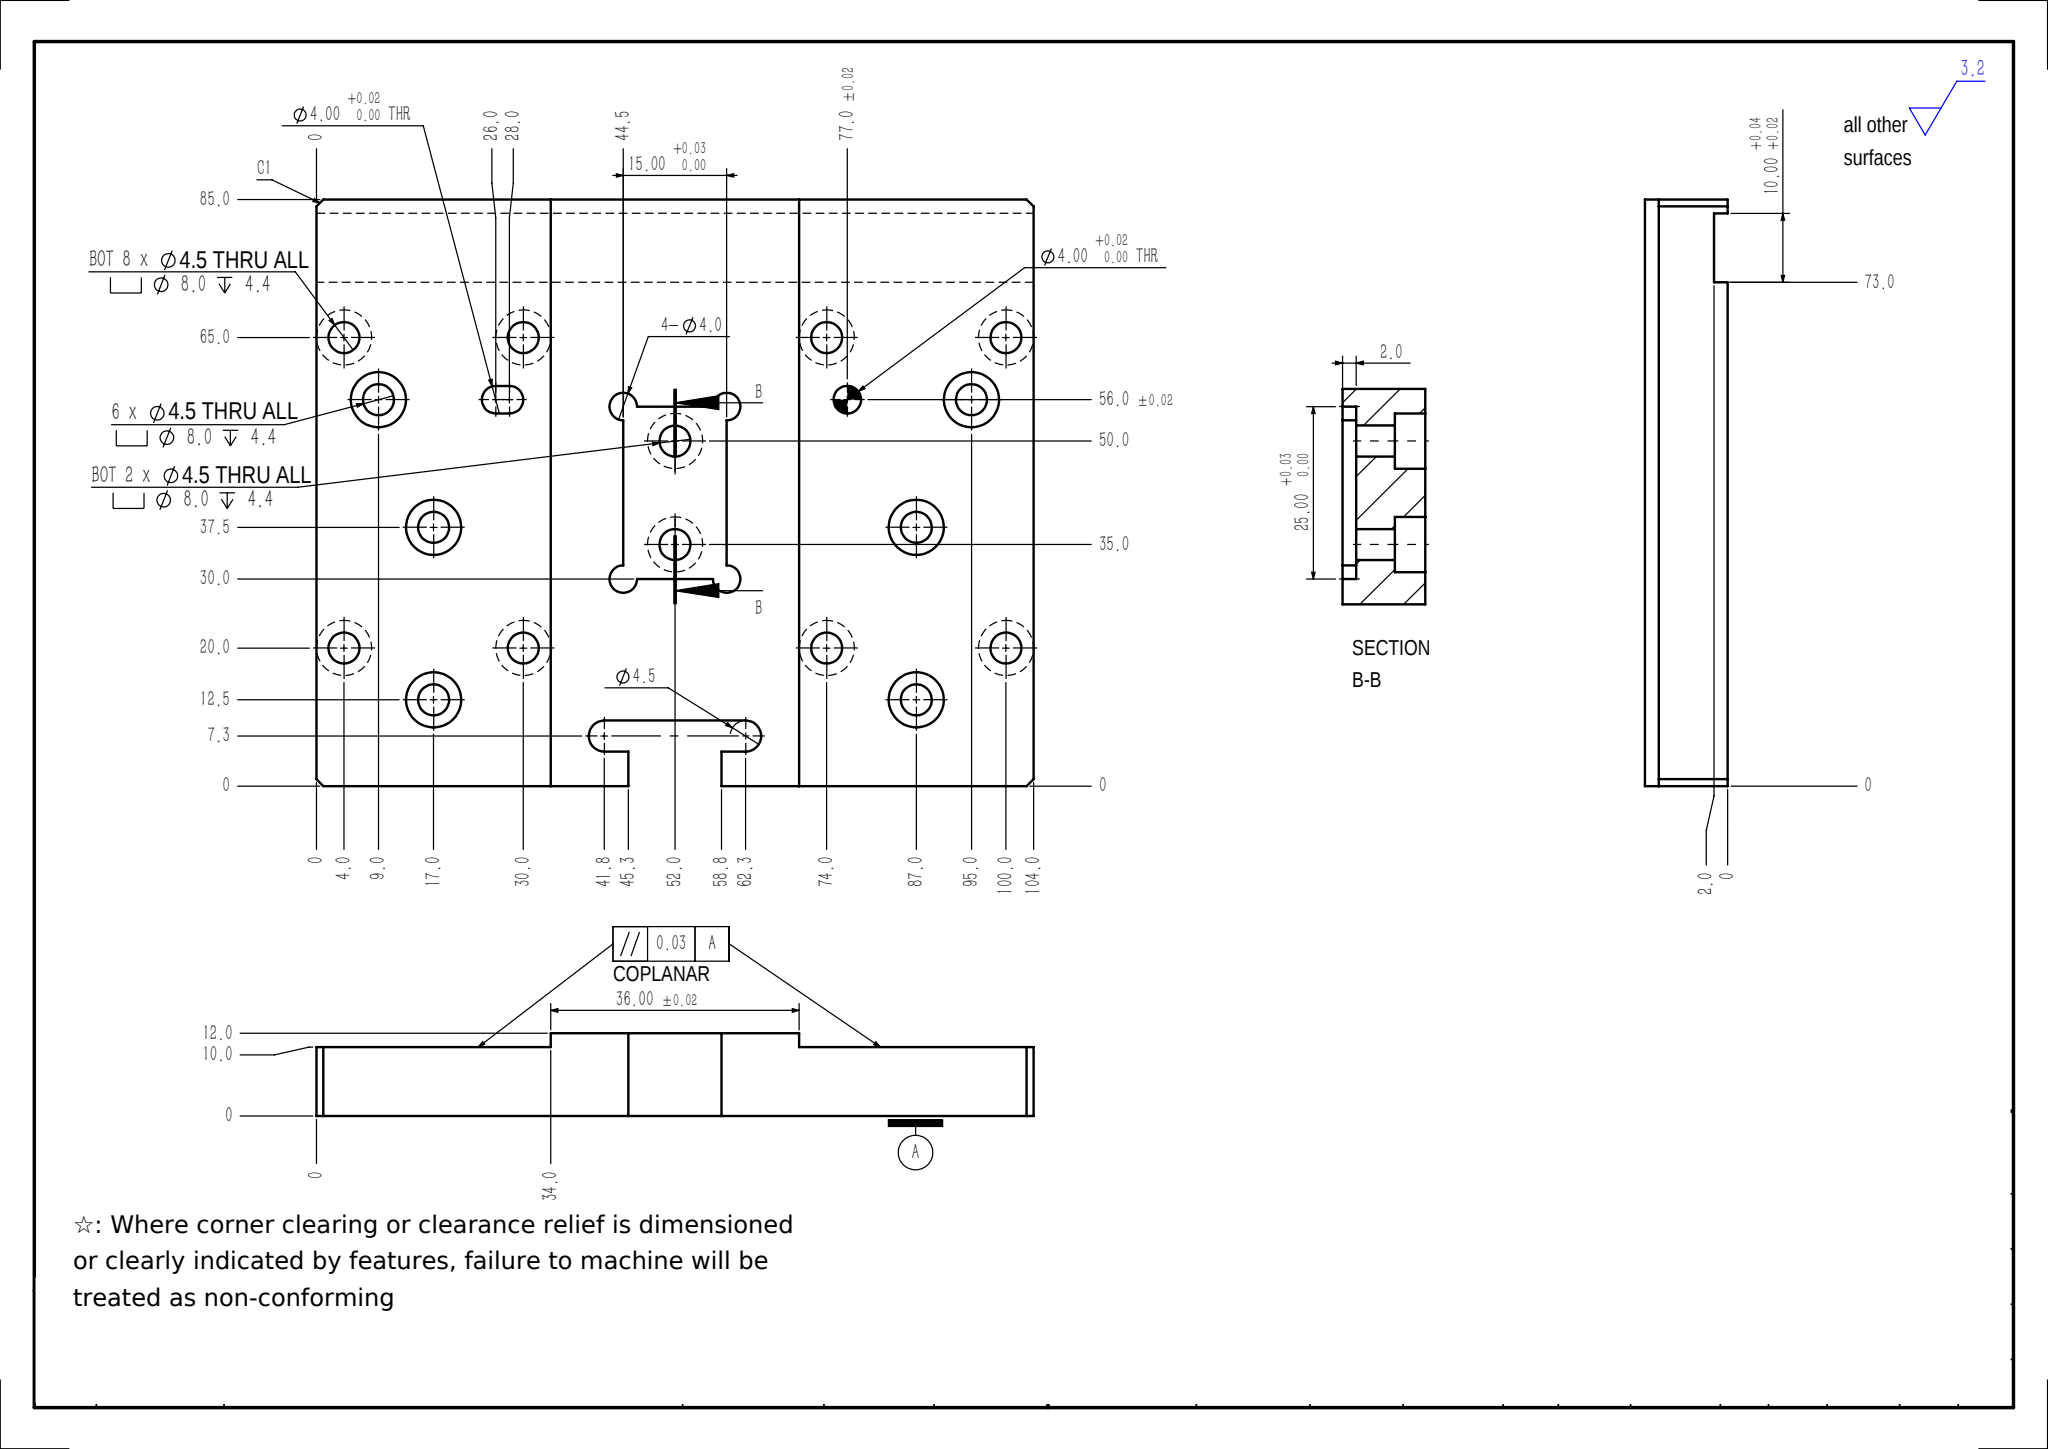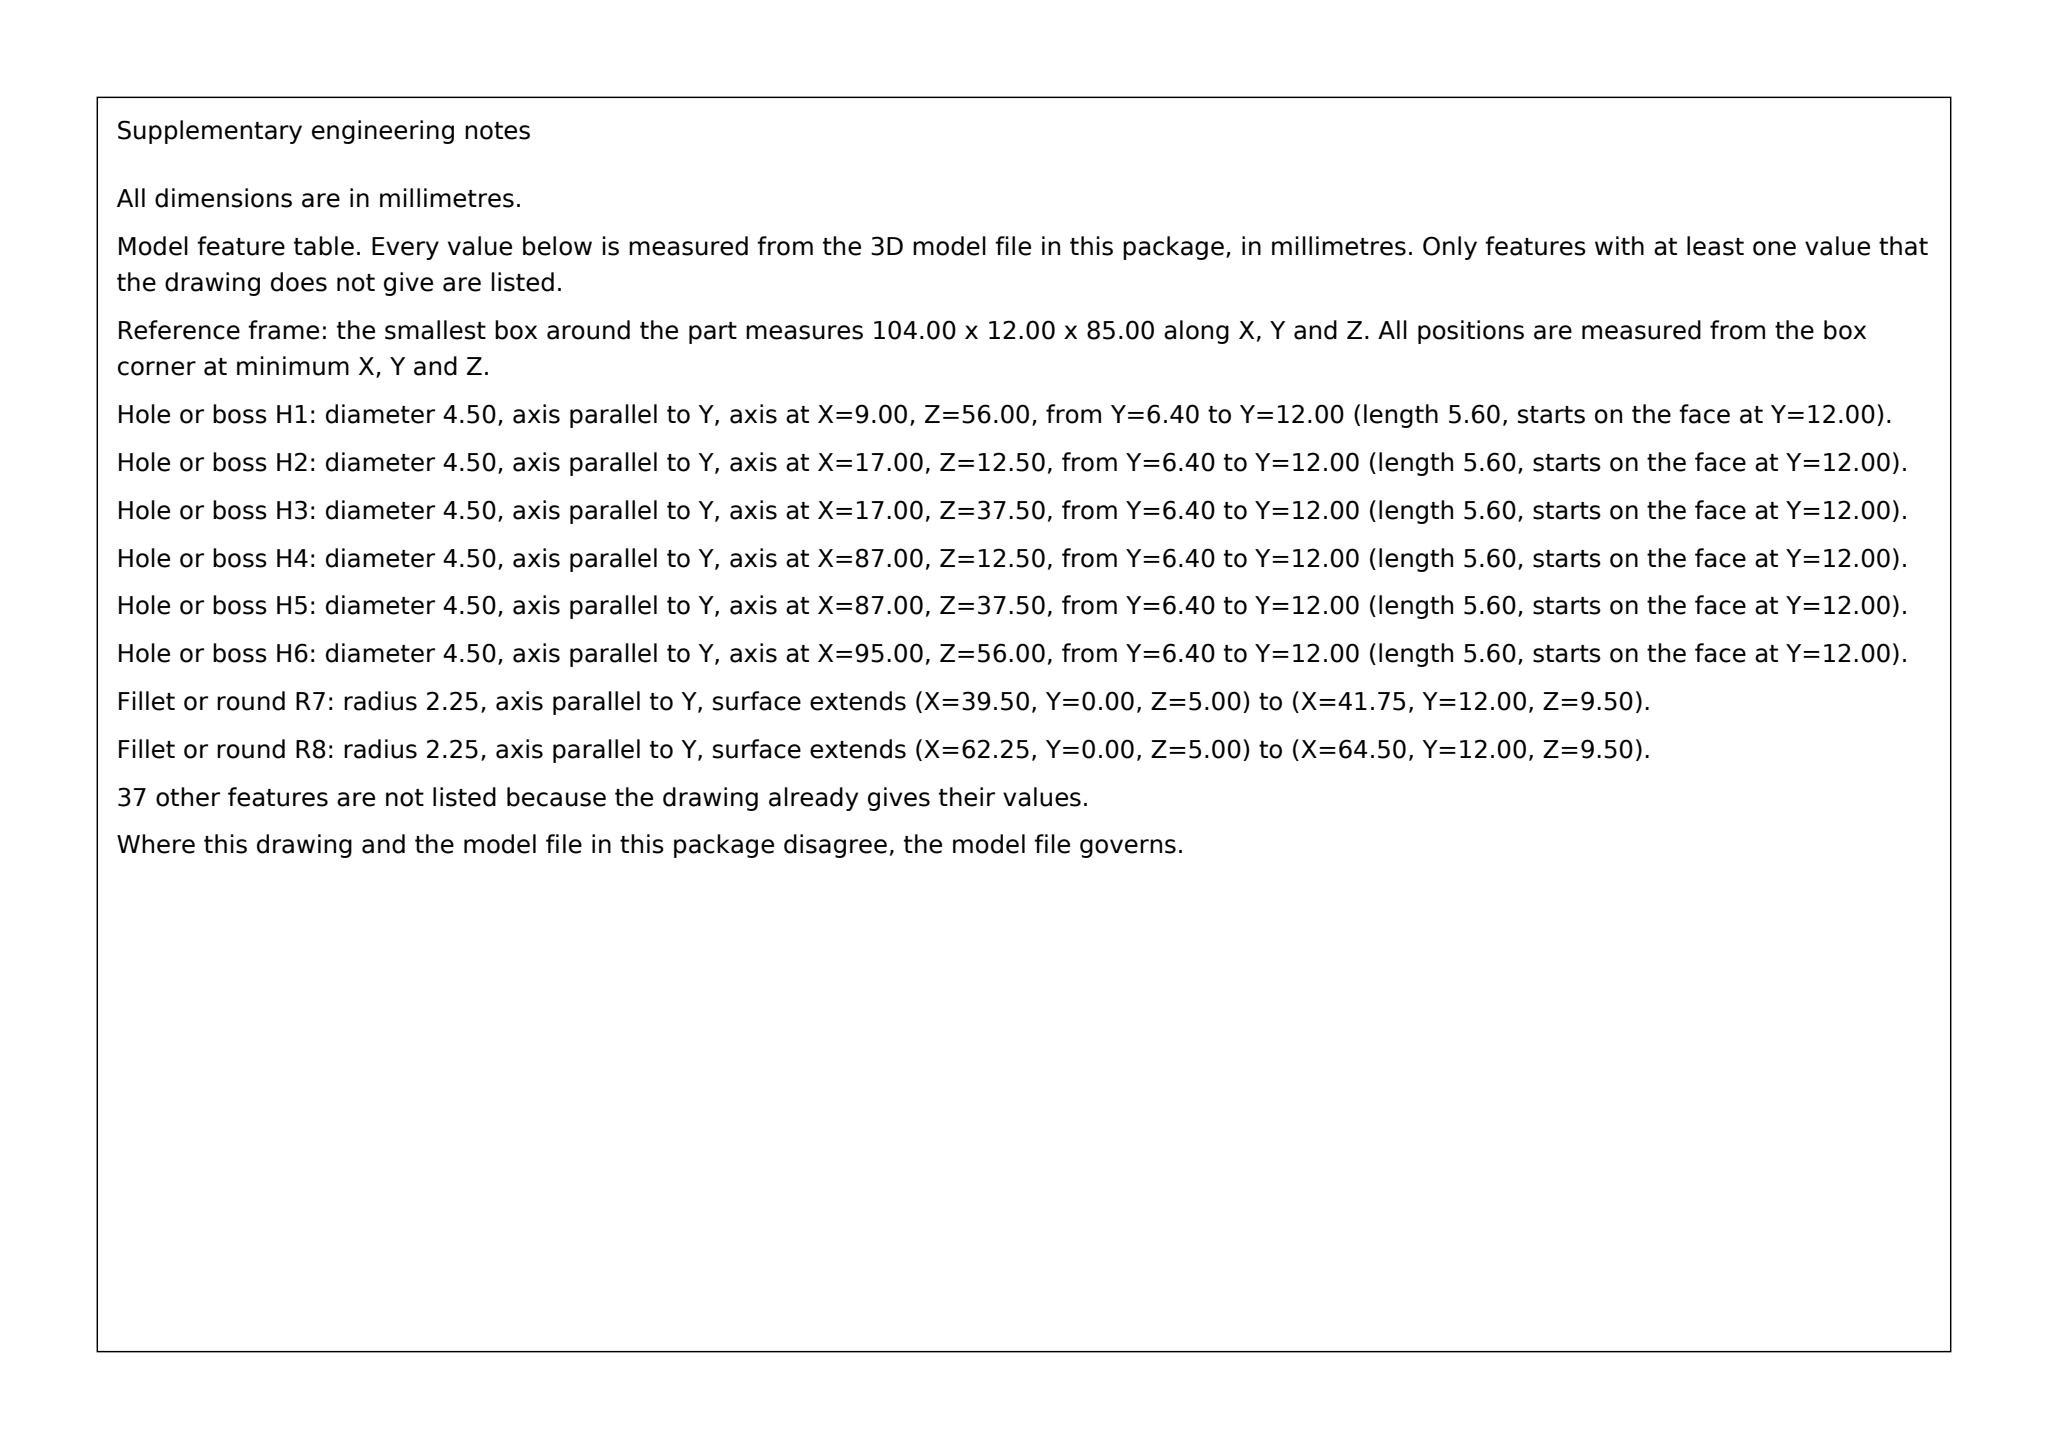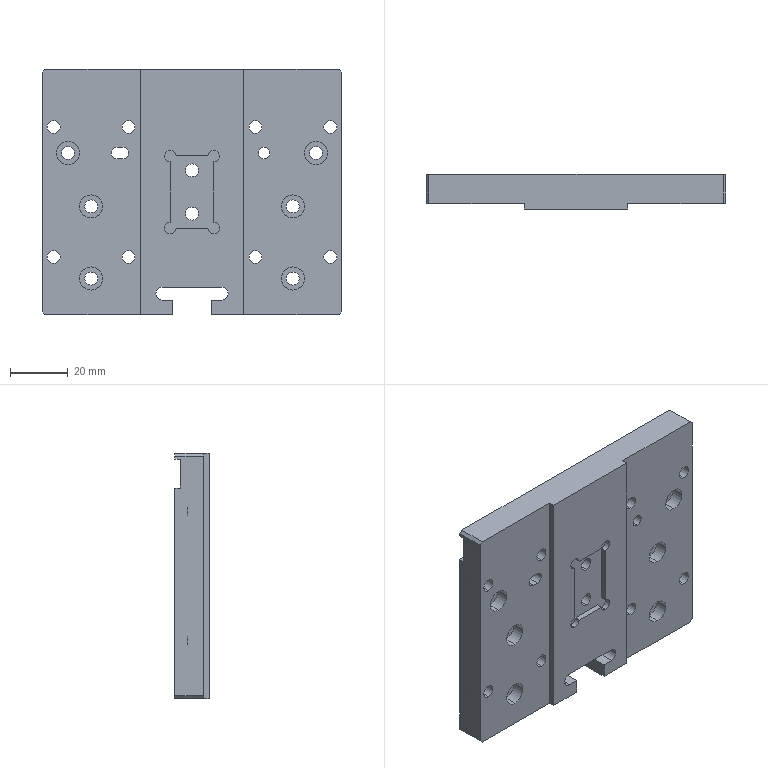Part | SolidWorks | mm | 1 solid | 125 faces | box 104 x 12 x 85 mm | volume 84192 mm3 | cylinder 78 | plane 47 | commonest cylinder face diameters 4.5 x36 8 x16 7.999 x16 4 x10